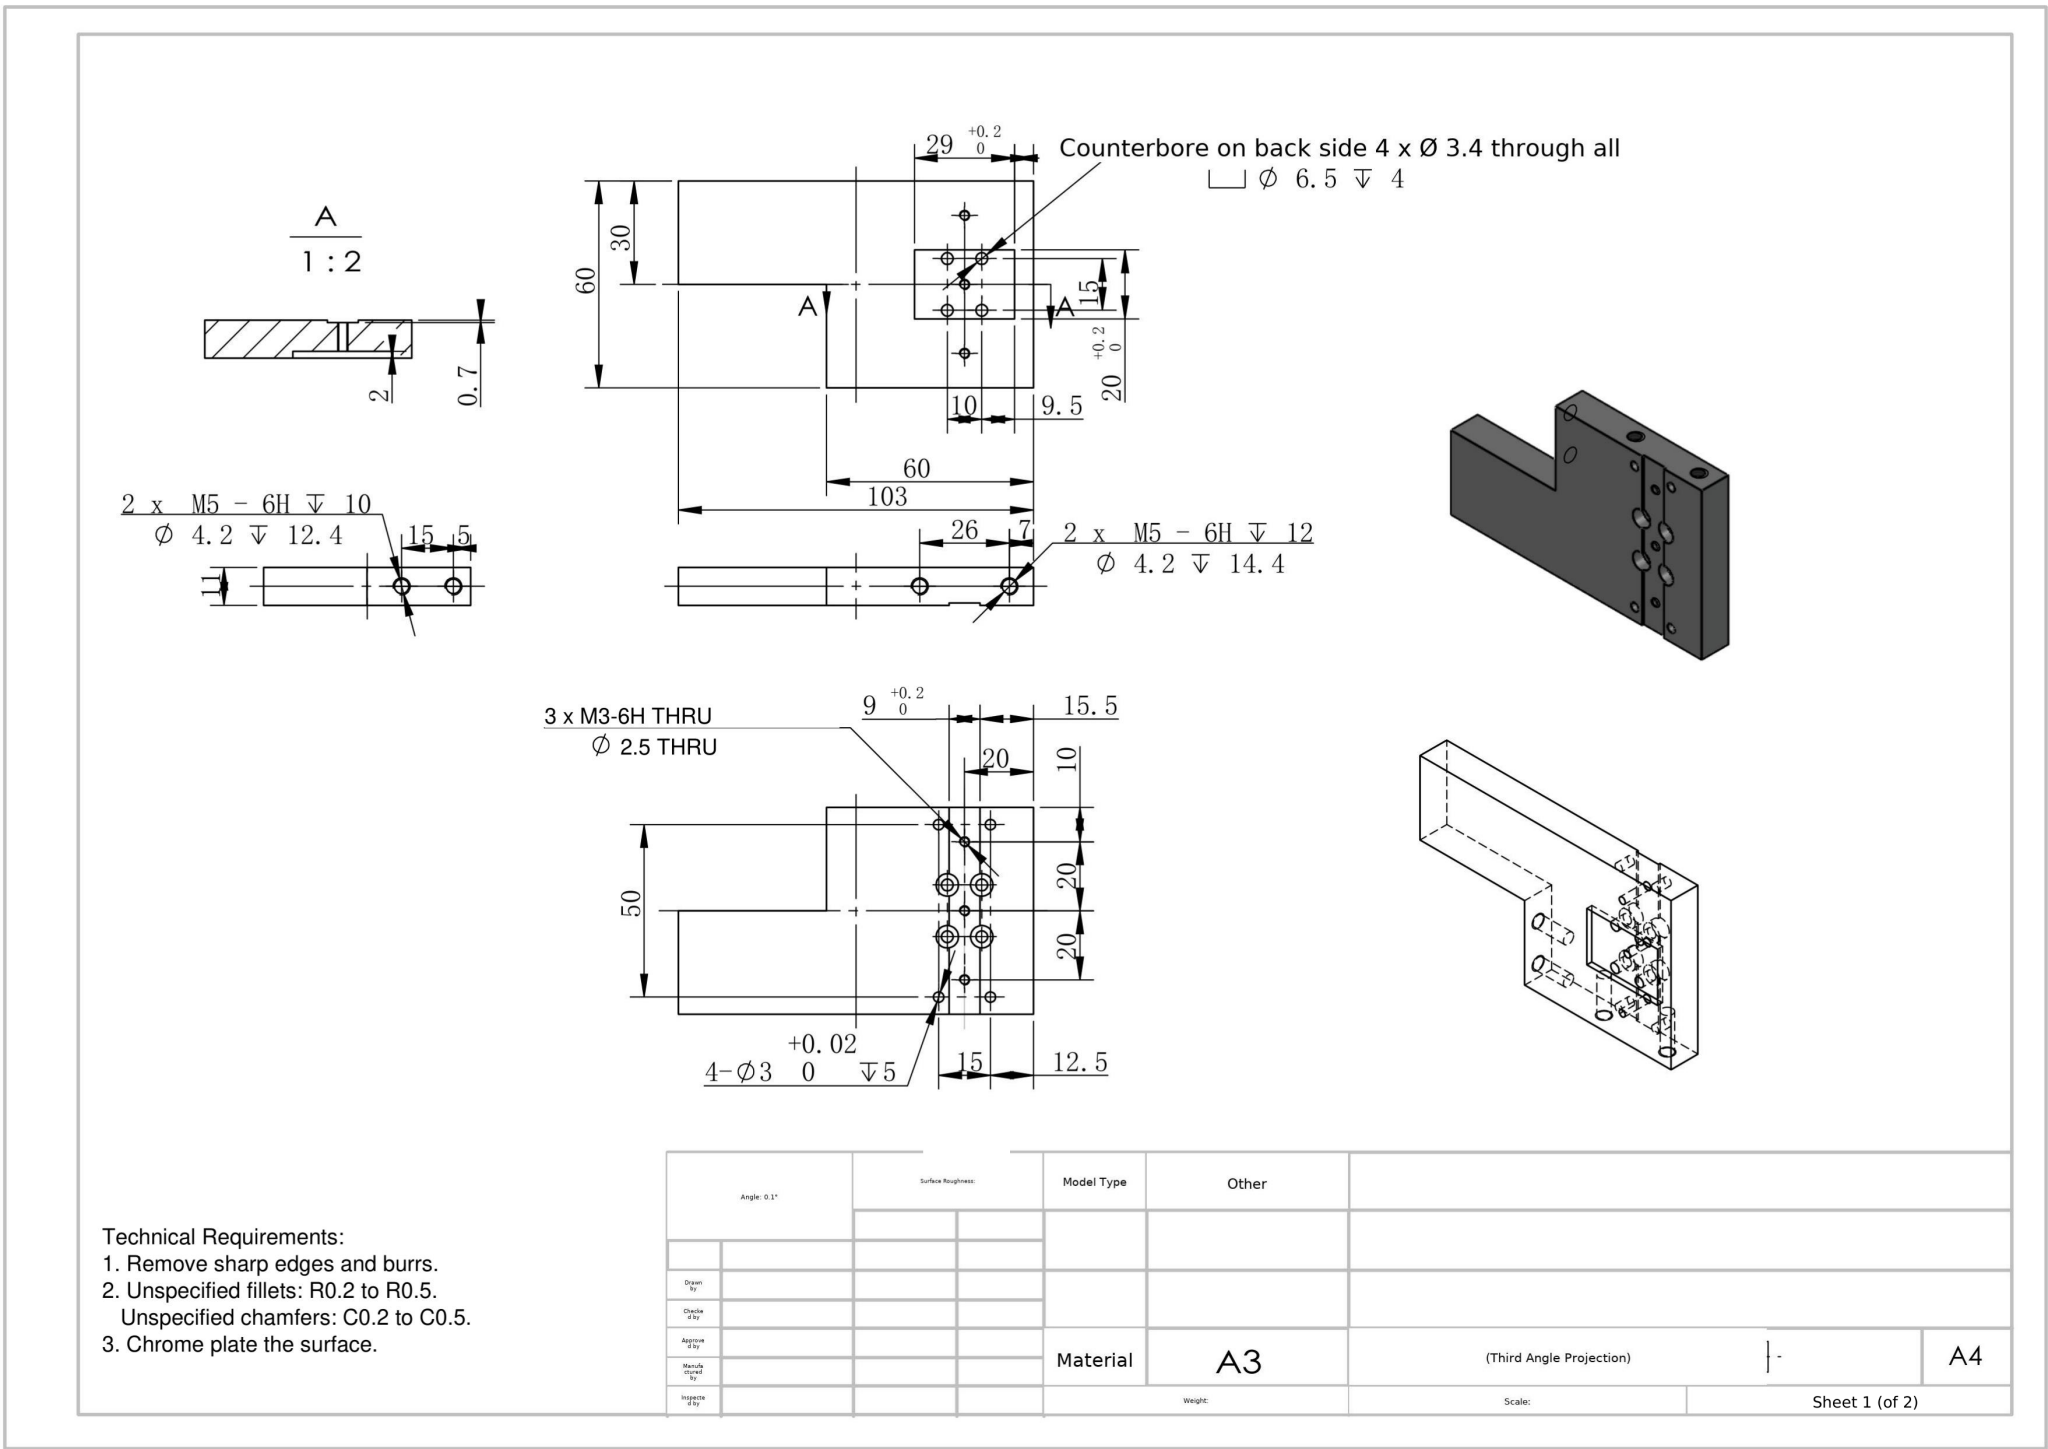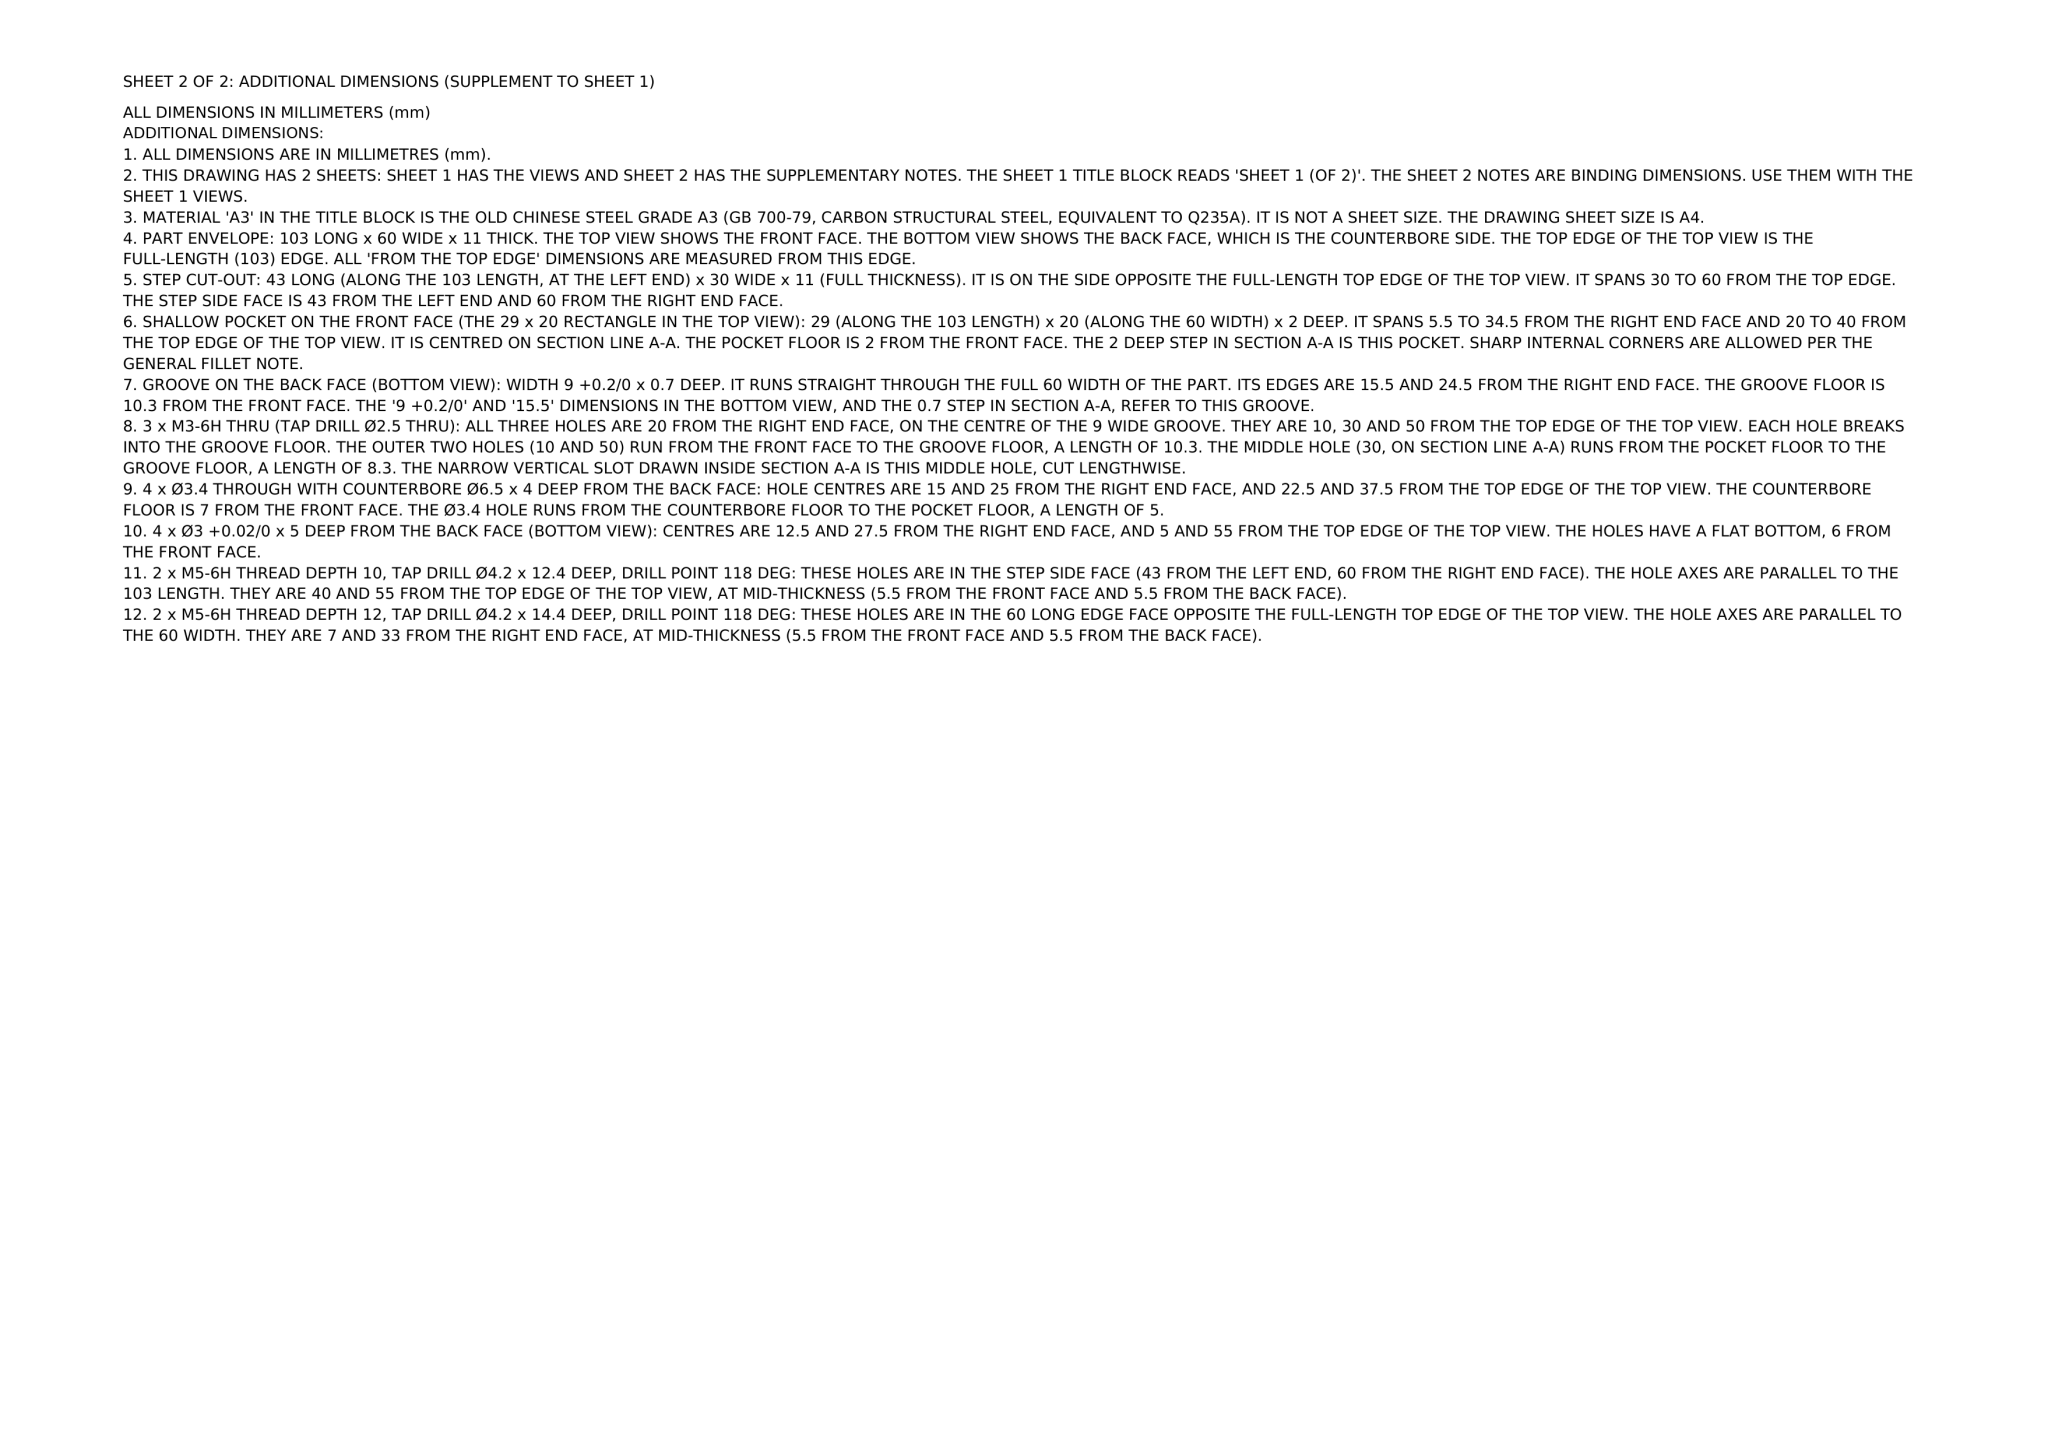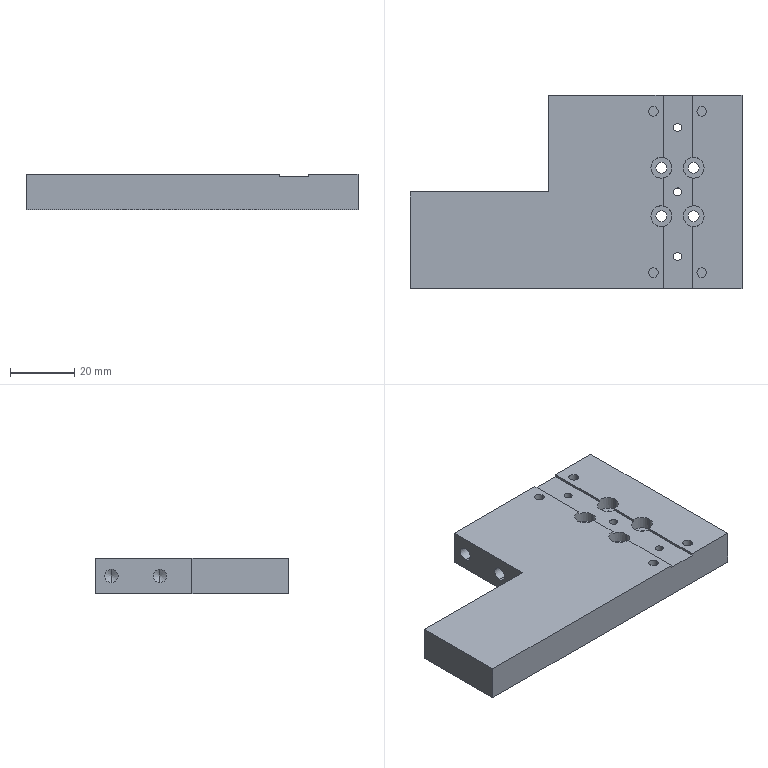Part | NX | mm | 1 solid | 75 faces | box 103 x 60 x 11 mm | volume 50528 mm3 | cylinder 38 | plane 29 | cone 8 | commonest cylinder face diameters 4.2 x8 3 x8 6.5 x8 3.4 x8 2.5 x6